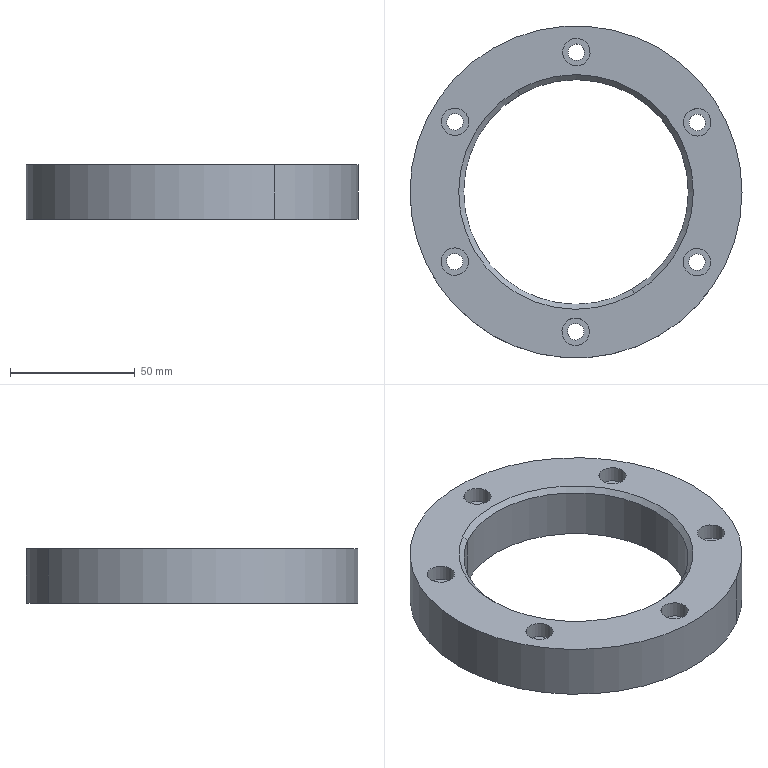Component | SolidWorks | ZN-A-020-1 | 1 solid | 38 faces | volume 158261 mm3 | cylinder 28 | plane 8 | cone 2 | commonest cylinder face diameters 11 x12 6.6 x12 90 x2 133 x2